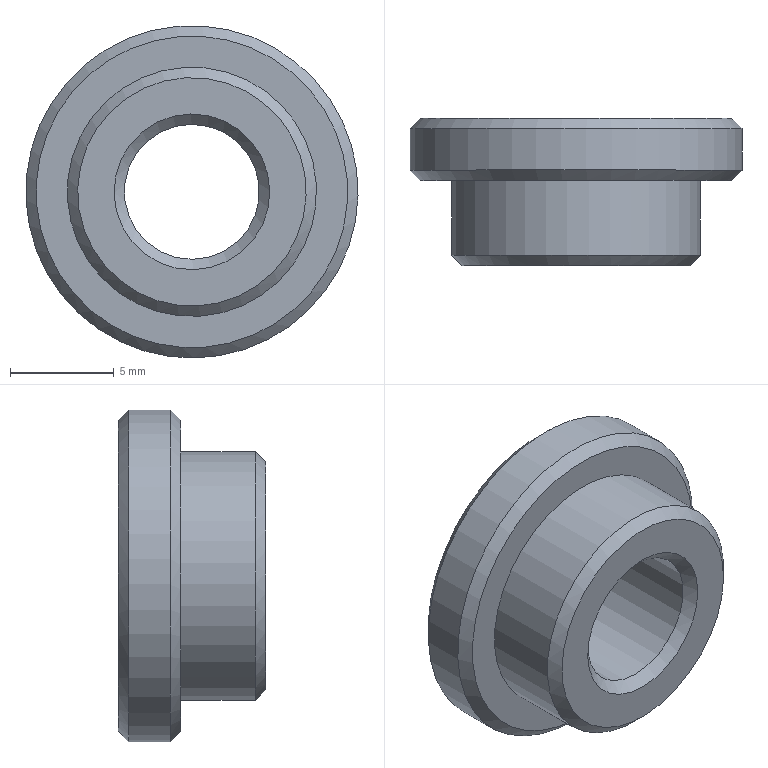Component | NX | BAFFLE | 1 solid | 10 faces | box 16 x 7.1 x 16 mm | volume 812 mm3 | cone 4 | plane 3 | cylinder 3 | commonest cylinder face diameters 16 x1 12 x1 6.5 x1
STEP:
#1=CARTESIAN_POINT('',(0.,0.,0.));
#2=DIRECTION('',(0.,0.,1.));
#3=DIRECTION('',(1.,0.,0.));
#4=AXIS2_PLACEMENT_3D('',#1,#2,#3);
#5=CARTESIAN_POINT('',(68.42,-2.,57.169));
#6=VERTEX_POINT('',#5);
#7=CARTESIAN_POINT('',(70.228,-2.,49.89));
#8=DIRECTION('',(0.,-1.,0.));
#9=DIRECTION('',(-0.2411,0.,0.9705));
#10=AXIS2_PLACEMENT_3D('',#7,#8,#9);
#11=CIRCLE('',#10,7.5);
#12=CARTESIAN_POINT('',(70.228,-2.,49.89));
#13=DIRECTION('',(0.,1.,0.));
#14=DIRECTION('',(-0.2411,0.,0.9705));
#15=AXIS2_PLACEMENT_3D('',#12,#13,#14);
#16=PLANE('',#15);
#17=CARTESIAN_POINT('',(7.5,0.));
#18=CARTESIAN_POINT('',(7.5,-12.99));
#19=CARTESIAN_POINT('',(-3.75,-6.495));
#20=CARTESIAN_POINT('',(-15.,-0.));
#21=CARTESIAN_POINT('',(-3.75,6.495));
#22=CARTESIAN_POINT('',(7.5,12.99));
#23=CARTESIAN_POINT('',(7.5,0.));
#24=(BOUNDED_CURVE()B_SPLINE_CURVE(2,(#17,#18,#19,#20,#21,#22,#23),.UNSPECIFIED.,.T.,.F.)B_SPLINE_CURVE_WITH_KNOTS((1,2,2,2,2,1),(-2.094,0.,2.094,4.189,6.283,8.378),.UNSPECIFIED.)CURVE()GEOMETRIC_REPRESENTATION_ITEM()RATIONAL_B_SPLINE_CURVE((1.,0.5,1.,0.5,1.,0.5,1.))REPRESENTATION_ITEM(''));
#25=(GEOMETRIC_REPRESENTATION_CONTEXT(2)PARAMETRIC_REPRESENTATION_CONTEXT()REPRESENTATION_CONTEXT('',''));
#26=DEFINITIONAL_REPRESENTATION('',(#24),#25);
#27=PCURVE('',#16,#26);
#28=CARTESIAN_POINT('',(70.228,-1.5,49.89));
#29=DIRECTION('',(0.,1.,0.));
#30=DIRECTION('',(-0.2411,0.,0.9705));
#31=AXIS2_PLACEMENT_3D('',#28,#29,#30);
#32=CONICAL_SURFACE('',#31,8.,0.7854);
#33=CARTESIAN_POINT('',(6.283,-0.5));
#34=DIRECTION('',(-1.,0.));
#35=VECTOR('',#34,1.);
#36=LINE('',#33,#35);
#37=(GEOMETRIC_REPRESENTATION_CONTEXT(2)PARAMETRIC_REPRESENTATION_CONTEXT()REPRESENTATION_CONTEXT('',''));
#38=DEFINITIONAL_REPRESENTATION('',(#36),#37);
#39=PCURVE('',#32,#38);
#40=SURFACE_CURVE('',#11,(#27,#39),.PCURVE_S1.);
#41=EDGE_CURVE('',#6,#6,#40,.T.);
#42=ORIENTED_EDGE('',*,*,#41,.T.);
#43=EDGE_LOOP('',(#42));
#44=FACE_BOUND('',#43,.T.);
#45=CARTESIAN_POINT('',(68.781,-2.,55.713));
#46=VERTEX_POINT('',#45);
#47=CARTESIAN_POINT('',(70.228,-2.,49.89));
#48=DIRECTION('',(0.,-1.,0.));
#49=DIRECTION('',(-0.2411,0.,0.9705));
#50=AXIS2_PLACEMENT_3D('',#47,#48,#49);
#51=CIRCLE('',#50,6.);
#52=CARTESIAN_POINT('',(6.,0.));
#53=CARTESIAN_POINT('',(6.,-10.392));
#54=CARTESIAN_POINT('',(-3.,-5.196));
#55=CARTESIAN_POINT('',(-12.,-0.));
#56=CARTESIAN_POINT('',(-3.,5.196));
#57=CARTESIAN_POINT('',(6.,10.392));
#58=CARTESIAN_POINT('',(6.,0.));
#59=(BOUNDED_CURVE()B_SPLINE_CURVE(2,(#52,#53,#54,#55,#56,#57,#58),.UNSPECIFIED.,.T.,.F.)B_SPLINE_CURVE_WITH_KNOTS((1,2,2,2,2,1),(-2.094,0.,2.094,4.189,6.283,8.378),.UNSPECIFIED.)CURVE()GEOMETRIC_REPRESENTATION_ITEM()RATIONAL_B_SPLINE_CURVE((1.,0.5,1.,0.5,1.,0.5,1.))REPRESENTATION_ITEM(''));
#60=(GEOMETRIC_REPRESENTATION_CONTEXT(2)PARAMETRIC_REPRESENTATION_CONTEXT()REPRESENTATION_CONTEXT('',''));
#61=DEFINITIONAL_REPRESENTATION('',(#59),#60);
#62=PCURVE('',#16,#61);
#63=CARTESIAN_POINT('',(70.228,-6.1,49.89));
#64=DIRECTION('',(0.,1.,0.));
#65=DIRECTION('',(-0.2411,0.,0.9705));
#66=AXIS2_PLACEMENT_3D('',#63,#64,#65);
#67=CYLINDRICAL_SURFACE('',#66,6.);
#68=CARTESIAN_POINT('',(6.283,4.1));
#69=DIRECTION('',(-1.,0.));
#70=VECTOR('',#69,1.);
#71=LINE('',#68,#70);
#72=(GEOMETRIC_REPRESENTATION_CONTEXT(2)PARAMETRIC_REPRESENTATION_CONTEXT()REPRESENTATION_CONTEXT('',''));
#73=DEFINITIONAL_REPRESENTATION('',(#71),#72);
#74=PCURVE('',#67,#73);
#75=SURFACE_CURVE('',#51,(#62,#74),.PCURVE_S1.);
#76=EDGE_CURVE('',#46,#46,#75,.T.);
#77=ORIENTED_EDGE('',*,*,#76,.F.);
#78=EDGE_LOOP('',(#77));
#79=FACE_BOUND('',#78,.T.);
#80=ADVANCED_FACE('',(#44,#79),#16,.F.);
#81=CARTESIAN_POINT('',(68.299,0.5,57.654));
#82=VERTEX_POINT('',#81);
#83=CARTESIAN_POINT('',(70.228,0.5,49.89));
#84=DIRECTION('',(0.,-1.,0.));
#85=DIRECTION('',(-0.2411,0.,0.9705));
#86=AXIS2_PLACEMENT_3D('',#83,#84,#85);
#87=CIRCLE('',#86,8.);
#88=CARTESIAN_POINT('',(70.228,1.,49.89));
#89=DIRECTION('',(0.,-1.,0.));
#90=DIRECTION('',(0.2411,0.,-0.9705));
#91=AXIS2_PLACEMENT_3D('',#88,#89,#90);
#92=CYLINDRICAL_SURFACE('',#91,8.);
#93=CARTESIAN_POINT('',(3.142,0.5));
#94=DIRECTION('',(1.,0.));
#95=VECTOR('',#94,1.);
#96=LINE('',#93,#95);
#97=(GEOMETRIC_REPRESENTATION_CONTEXT(2)PARAMETRIC_REPRESENTATION_CONTEXT()REPRESENTATION_CONTEXT('',''));
#98=DEFINITIONAL_REPRESENTATION('',(#96),#97);
#99=PCURVE('',#92,#98);
#100=CARTESIAN_POINT('',(70.228,1.,49.89));
#101=DIRECTION('',(0.,-1.,0.));
#102=DIRECTION('',(0.2411,0.,-0.9705));
#103=AXIS2_PLACEMENT_3D('',#100,#101,#102);
#104=CONICAL_SURFACE('',#103,7.5,0.7854);
#105=CARTESIAN_POINT('',(3.142,0.5));
#106=DIRECTION('',(1.,0.));
#107=VECTOR('',#106,1.);
#108=LINE('',#105,#107);
#109=(GEOMETRIC_REPRESENTATION_CONTEXT(2)PARAMETRIC_REPRESENTATION_CONTEXT()REPRESENTATION_CONTEXT('',''));
#110=DEFINITIONAL_REPRESENTATION('',(#108),#109);
#111=PCURVE('',#104,#110);
#112=SURFACE_CURVE('',#87,(#99,#111),.PCURVE_S1.);
#113=EDGE_CURVE('',#82,#82,#112,.T.);
#114=ORIENTED_EDGE('',*,*,#113,.T.);
#115=CARTESIAN_POINT('',(68.299,-1.5,57.654));
#116=VERTEX_POINT('',#115);
#117=CARTESIAN_POINT('',(68.299,0.5,57.654));
#118=CARTESIAN_POINT('',(68.299,-1.5,57.654));
#119=B_SPLINE_CURVE_WITH_KNOTS('',1,(#117,#118),.UNSPECIFIED.,.F.,.F.,(2,2),(0.5,2.5),.PIECEWISE_BEZIER_KNOTS.);
#120=CARTESIAN_POINT('',(9.425,0.));
#121=DIRECTION('',(0.,1.));
#122=VECTOR('',#121,1.);
#123=LINE('',#120,#122);
#124=(GEOMETRIC_REPRESENTATION_CONTEXT(2)PARAMETRIC_REPRESENTATION_CONTEXT()REPRESENTATION_CONTEXT('',''));
#125=DEFINITIONAL_REPRESENTATION('',(#123),#124);
#126=PCURVE('',#92,#125);
#127=CARTESIAN_POINT('',(3.142,0.));
#128=DIRECTION('',(0.,1.));
#129=VECTOR('',#128,1.);
#130=LINE('',#127,#129);
#131=(GEOMETRIC_REPRESENTATION_CONTEXT(2)PARAMETRIC_REPRESENTATION_CONTEXT()REPRESENTATION_CONTEXT('',''));
#132=DEFINITIONAL_REPRESENTATION('',(#130),#131);
#133=PCURVE('',#92,#132);
#134=SEAM_CURVE('',#119,(#126,#133),.PCURVE_S1.);
#135=EDGE_CURVE('',#82,#116,#134,.T.);
#136=ORIENTED_EDGE('',*,*,#135,.T.);
#137=CARTESIAN_POINT('',(70.228,-1.5,49.89));
#138=DIRECTION('',(0.,1.,0.));
#139=DIRECTION('',(-0.2411,0.,0.9705));
#140=AXIS2_PLACEMENT_3D('',#137,#138,#139);
#141=CIRCLE('',#140,8.);
#142=CARTESIAN_POINT('',(9.425,2.5));
#143=DIRECTION('',(-1.,0.));
#144=VECTOR('',#143,1.);
#145=LINE('',#142,#144);
#146=(GEOMETRIC_REPRESENTATION_CONTEXT(2)PARAMETRIC_REPRESENTATION_CONTEXT()REPRESENTATION_CONTEXT('',''));
#147=DEFINITIONAL_REPRESENTATION('',(#145),#146);
#148=PCURVE('',#92,#147);
#149=CARTESIAN_POINT('',(0.,0.));
#150=DIRECTION('',(1.,0.));
#151=VECTOR('',#150,1.);
#152=LINE('',#149,#151);
#153=(GEOMETRIC_REPRESENTATION_CONTEXT(2)PARAMETRIC_REPRESENTATION_CONTEXT()REPRESENTATION_CONTEXT('',''));
#154=DEFINITIONAL_REPRESENTATION('',(#152),#153);
#155=PCURVE('',#32,#154);
#156=SURFACE_CURVE('',#141,(#148,#155),.PCURVE_S1.);
#157=EDGE_CURVE('',#116,#116,#156,.T.);
#158=ORIENTED_EDGE('',*,*,#157,.T.);
#159=ORIENTED_EDGE('',*,*,#135,.F.);
#160=EDGE_LOOP('',(#114,#136,#158,#159));
#161=FACE_BOUND('',#160,.T.);
#162=ADVANCED_FACE('',(#161),#92,.T.);
#163=CARTESIAN_POINT('',(68.42,1.,57.169));
#164=VERTEX_POINT('',#163);
#165=CARTESIAN_POINT('',(70.228,1.,49.89));
#166=DIRECTION('',(0.,1.,0.));
#167=DIRECTION('',(-0.2411,0.,0.9705));
#168=AXIS2_PLACEMENT_3D('',#165,#166,#167);
#169=CIRCLE('',#168,7.5);
#170=CARTESIAN_POINT('',(70.228,1.,49.89));
#171=DIRECTION('',(0.,1.,0.));
#172=DIRECTION('',(-0.2411,0.,0.9705));
#173=AXIS2_PLACEMENT_3D('',#170,#171,#172);
#174=PLANE('',#173);
#175=CARTESIAN_POINT('',(0.,0.));
#176=DIRECTION('',(1.,0.));
#177=AXIS2_PLACEMENT_2D('',#175,#176);
#178=CIRCLE('',#177,7.5);
#179=(GEOMETRIC_REPRESENTATION_CONTEXT(2)PARAMETRIC_REPRESENTATION_CONTEXT()REPRESENTATION_CONTEXT('',''));
#180=DEFINITIONAL_REPRESENTATION('',(#178),#179);
#181=PCURVE('',#174,#180);
#182=CARTESIAN_POINT('',(9.425,0.));
#183=DIRECTION('',(-1.,0.));
#184=VECTOR('',#183,1.);
#185=LINE('',#182,#184);
#186=(GEOMETRIC_REPRESENTATION_CONTEXT(2)PARAMETRIC_REPRESENTATION_CONTEXT()REPRESENTATION_CONTEXT('',''));
#187=DEFINITIONAL_REPRESENTATION('',(#185),#186);
#188=PCURVE('',#104,#187);
#189=SURFACE_CURVE('',#169,(#181,#188),.PCURVE_S1.);
#190=EDGE_CURVE('',#164,#164,#189,.T.);
#191=ORIENTED_EDGE('',*,*,#190,.T.);
#192=EDGE_LOOP('',(#191));
#193=FACE_BOUND('',#192,.T.);
#194=CARTESIAN_POINT('',(69.444,1.,53.044));
#195=VERTEX_POINT('',#194);
#196=CARTESIAN_POINT('',(70.228,1.,49.89));
#197=DIRECTION('',(0.,1.,0.));
#198=DIRECTION('',(-0.2411,0.,0.9705));
#199=AXIS2_PLACEMENT_3D('',#196,#197,#198);
#200=CIRCLE('',#199,3.25);
#201=CARTESIAN_POINT('',(0.,0.));
#202=DIRECTION('',(1.,-0.));
#203=AXIS2_PLACEMENT_2D('',#201,#202);
#204=CIRCLE('',#203,3.25);
#205=(GEOMETRIC_REPRESENTATION_CONTEXT(2)PARAMETRIC_REPRESENTATION_CONTEXT()REPRESENTATION_CONTEXT('',''));
#206=DEFINITIONAL_REPRESENTATION('',(#204),#205);
#207=PCURVE('',#174,#206);
#208=CARTESIAN_POINT('',(70.228,-6.1,49.89));
#209=DIRECTION('',(0.,1.,0.));
#210=DIRECTION('',(-0.2411,0.,0.9705));
#211=AXIS2_PLACEMENT_3D('',#208,#209,#210);
#212=CYLINDRICAL_SURFACE('',#211,3.25);
#213=CARTESIAN_POINT('',(0.,7.1));
#214=DIRECTION('',(1.,0.));
#215=VECTOR('',#214,1.);
#216=LINE('',#213,#215);
#217=(GEOMETRIC_REPRESENTATION_CONTEXT(2)PARAMETRIC_REPRESENTATION_CONTEXT()REPRESENTATION_CONTEXT('',''));
#218=DEFINITIONAL_REPRESENTATION('',(#216),#217);
#219=PCURVE('',#212,#218);
#220=SURFACE_CURVE('',#200,(#207,#219),.PCURVE_S1.);
#221=EDGE_CURVE('',#195,#195,#220,.T.);
#222=ORIENTED_EDGE('',*,*,#221,.F.);
#223=EDGE_LOOP('',(#222));
#224=FACE_BOUND('',#223,.T.);
#225=ADVANCED_FACE('',(#193,#224),#174,.T.);
#226=CARTESIAN_POINT('',(71.674,-5.6,44.067));
#227=VERTEX_POINT('',#226);
#228=CARTESIAN_POINT('',(68.781,-5.6,55.713));
#229=VERTEX_POINT('',#228);
#230=CARTESIAN_POINT('',(70.228,-5.6,49.89));
#231=DIRECTION('',(0.,1.,0.));
#232=DIRECTION('',(0.2411,0.,-0.9705));
#233=AXIS2_PLACEMENT_3D('',#230,#231,#232);
#234=CIRCLE('',#233,6.);
#235=CARTESIAN_POINT('',(3.142,0.5));
#236=DIRECTION('',(1.,0.));
#237=VECTOR('',#236,1.);
#238=LINE('',#235,#237);
#239=(GEOMETRIC_REPRESENTATION_CONTEXT(2)PARAMETRIC_REPRESENTATION_CONTEXT()REPRESENTATION_CONTEXT('',''));
#240=DEFINITIONAL_REPRESENTATION('',(#238),#239);
#241=PCURVE('',#67,#240);
#242=CARTESIAN_POINT('',(70.228,-6.1,49.89));
#243=DIRECTION('',(0.,1.,0.));
#244=DIRECTION('',(-0.2411,0.,0.9705));
#245=AXIS2_PLACEMENT_3D('',#242,#243,#244);
#246=CONICAL_SURFACE('',#245,5.5,0.7854);
#247=CARTESIAN_POINT('',(3.142,0.5));
#248=DIRECTION('',(1.,-0.));
#249=VECTOR('',#248,1.);
#250=LINE('',#247,#249);
#251=(GEOMETRIC_REPRESENTATION_CONTEXT(2)PARAMETRIC_REPRESENTATION_CONTEXT()REPRESENTATION_CONTEXT('',''));
#252=DEFINITIONAL_REPRESENTATION('',(#250),#251);
#253=PCURVE('',#246,#252);
#254=SURFACE_CURVE('',#234,(#241,#253),.PCURVE_S1.);
#255=EDGE_CURVE('',#227,#229,#254,.T.);
#256=ORIENTED_EDGE('',*,*,#255,.T.);
#257=CARTESIAN_POINT('',(68.781,-5.6,55.713));
#258=CARTESIAN_POINT('',(68.781,-2.,55.713));
#259=B_SPLINE_CURVE_WITH_KNOTS('',1,(#257,#258),.UNSPECIFIED.,.F.,.F.,(2,2),(0.5,4.1),.PIECEWISE_BEZIER_KNOTS.);
#260=CARTESIAN_POINT('',(6.283,0.));
#261=DIRECTION('',(0.,1.));
#262=VECTOR('',#261,1.);
#263=LINE('',#260,#262);
#264=(GEOMETRIC_REPRESENTATION_CONTEXT(2)PARAMETRIC_REPRESENTATION_CONTEXT()REPRESENTATION_CONTEXT('',''));
#265=DEFINITIONAL_REPRESENTATION('',(#263),#264);
#266=PCURVE('',#67,#265);
#267=CARTESIAN_POINT('',(0.,0.));
#268=DIRECTION('',(0.,1.));
#269=VECTOR('',#268,1.);
#270=LINE('',#267,#269);
#271=(GEOMETRIC_REPRESENTATION_CONTEXT(2)PARAMETRIC_REPRESENTATION_CONTEXT()REPRESENTATION_CONTEXT('',''));
#272=DEFINITIONAL_REPRESENTATION('',(#270),#271);
#273=PCURVE('',#67,#272);
#274=SEAM_CURVE('',#259,(#266,#273),.PCURVE_S1.);
#275=EDGE_CURVE('',#229,#46,#274,.T.);
#276=ORIENTED_EDGE('',*,*,#275,.T.);
#277=ORIENTED_EDGE('',*,*,#76,.T.);
#278=ORIENTED_EDGE('',*,*,#275,.F.);
#279=CARTESIAN_POINT('',(70.228,-5.6,49.89));
#280=DIRECTION('',(0.,1.,0.));
#281=DIRECTION('',(0.2411,0.,-0.9705));
#282=AXIS2_PLACEMENT_3D('',#279,#280,#281);
#283=CIRCLE('',#282,6.);
#284=CARTESIAN_POINT('',(-3.142,0.5));
#285=DIRECTION('',(1.,0.));
#286=VECTOR('',#285,1.);
#287=LINE('',#284,#286);
#288=(GEOMETRIC_REPRESENTATION_CONTEXT(2)PARAMETRIC_REPRESENTATION_CONTEXT()REPRESENTATION_CONTEXT('',''));
#289=DEFINITIONAL_REPRESENTATION('',(#287),#288);
#290=PCURVE('',#67,#289);
#291=CARTESIAN_POINT('',(3.142,0.5));
#292=DIRECTION('',(1.,0.));
#293=VECTOR('',#292,1.);
#294=LINE('',#291,#293);
#295=(GEOMETRIC_REPRESENTATION_CONTEXT(2)PARAMETRIC_REPRESENTATION_CONTEXT()REPRESENTATION_CONTEXT('',''));
#296=DEFINITIONAL_REPRESENTATION('',(#294),#295);
#297=PCURVE('',#246,#296);
#298=SURFACE_CURVE('',#283,(#290,#297),.PCURVE_S1.);
#299=EDGE_CURVE('',#229,#227,#298,.T.);
#300=ORIENTED_EDGE('',*,*,#299,.T.);
#301=EDGE_LOOP('',(#256,#276,#277,#278,#300));
#302=FACE_BOUND('',#301,.T.);
#303=ADVANCED_FACE('',(#302),#67,.T.);
#304=CARTESIAN_POINT('',(69.444,-5.6,53.044));
#305=VERTEX_POINT('',#304);
#306=CARTESIAN_POINT('',(71.011,-5.6,46.736));
#307=VERTEX_POINT('',#306);
#308=CARTESIAN_POINT('',(70.228,-5.6,49.89));
#309=DIRECTION('',(0.,-1.,0.));
#310=DIRECTION('',(0.2411,0.,-0.9705));
#311=AXIS2_PLACEMENT_3D('',#308,#309,#310);
#312=CIRCLE('',#311,3.25);
#313=CARTESIAN_POINT('',(9.425,0.5));
#314=DIRECTION('',(-1.,0.));
#315=VECTOR('',#314,1.);
#316=LINE('',#313,#315);
#317=(GEOMETRIC_REPRESENTATION_CONTEXT(2)PARAMETRIC_REPRESENTATION_CONTEXT()REPRESENTATION_CONTEXT('',''));
#318=DEFINITIONAL_REPRESENTATION('',(#316),#317);
#319=PCURVE('',#212,#318);
#320=CARTESIAN_POINT('',(70.228,-6.1,49.89));
#321=DIRECTION('',(0.,-1.,0.));
#322=DIRECTION('',(0.2411,0.,-0.9705));
#323=AXIS2_PLACEMENT_3D('',#320,#321,#322);
#324=CONICAL_SURFACE('',#323,3.75,0.7854);
#325=CARTESIAN_POINT('',(0.,-0.5));
#326=DIRECTION('',(1.,-0.));
#327=VECTOR('',#326,1.);
#328=LINE('',#325,#327);
#329=(GEOMETRIC_REPRESENTATION_CONTEXT(2)PARAMETRIC_REPRESENTATION_CONTEXT()REPRESENTATION_CONTEXT('',''));
#330=DEFINITIONAL_REPRESENTATION('',(#328),#329);
#331=PCURVE('',#324,#330);
#332=SURFACE_CURVE('',#312,(#319,#331),.PCURVE_S1.);
#333=EDGE_CURVE('',#305,#307,#332,.T.);
#334=ORIENTED_EDGE('',*,*,#333,.F.);
#335=CARTESIAN_POINT('',(69.444,-5.6,53.044));
#336=CARTESIAN_POINT('',(69.444,1.,53.044));
#337=B_SPLINE_CURVE_WITH_KNOTS('',1,(#335,#336),.UNSPECIFIED.,.F.,.F.,(2,2),(0.5,7.1),.PIECEWISE_BEZIER_KNOTS.);
#338=CARTESIAN_POINT('',(6.283,0.));
#339=DIRECTION('',(0.,1.));
#340=VECTOR('',#339,1.);
#341=LINE('',#338,#340);
#342=(GEOMETRIC_REPRESENTATION_CONTEXT(2)PARAMETRIC_REPRESENTATION_CONTEXT()REPRESENTATION_CONTEXT('',''));
#343=DEFINITIONAL_REPRESENTATION('',(#341),#342);
#344=PCURVE('',#212,#343);
#345=CARTESIAN_POINT('',(0.,0.));
#346=DIRECTION('',(0.,1.));
#347=VECTOR('',#346,1.);
#348=LINE('',#345,#347);
#349=(GEOMETRIC_REPRESENTATION_CONTEXT(2)PARAMETRIC_REPRESENTATION_CONTEXT()REPRESENTATION_CONTEXT('',''));
#350=DEFINITIONAL_REPRESENTATION('',(#348),#349);
#351=PCURVE('',#212,#350);
#352=SEAM_CURVE('',#337,(#344,#351),.PCURVE_S1.);
#353=EDGE_CURVE('',#305,#195,#352,.T.);
#354=ORIENTED_EDGE('',*,*,#353,.T.);
#355=ORIENTED_EDGE('',*,*,#221,.F.);
#356=ORIENTED_EDGE('',*,*,#353,.F.);
#357=CARTESIAN_POINT('',(70.228,-5.6,49.89));
#358=DIRECTION('',(0.,-1.,0.));
#359=DIRECTION('',(0.2411,0.,-0.9705));
#360=AXIS2_PLACEMENT_3D('',#357,#358,#359);
#361=CIRCLE('',#360,3.25);
#362=CARTESIAN_POINT('',(3.142,0.5));
#363=DIRECTION('',(-1.,0.));
#364=VECTOR('',#363,1.);
#365=LINE('',#362,#364);
#366=(GEOMETRIC_REPRESENTATION_CONTEXT(2)PARAMETRIC_REPRESENTATION_CONTEXT()REPRESENTATION_CONTEXT('',''));
#367=DEFINITIONAL_REPRESENTATION('',(#365),#366);
#368=PCURVE('',#212,#367);
#369=CARTESIAN_POINT('',(0.,-0.5));
#370=DIRECTION('',(1.,0.));
#371=VECTOR('',#370,1.);
#372=LINE('',#369,#371);
#373=(GEOMETRIC_REPRESENTATION_CONTEXT(2)PARAMETRIC_REPRESENTATION_CONTEXT()REPRESENTATION_CONTEXT('',''));
#374=DEFINITIONAL_REPRESENTATION('',(#372),#373);
#375=PCURVE('',#324,#374);
#376=SURFACE_CURVE('',#361,(#368,#375),.PCURVE_S1.);
#377=EDGE_CURVE('',#307,#305,#376,.T.);
#378=ORIENTED_EDGE('',*,*,#377,.F.);
#379=EDGE_LOOP('',(#334,#354,#355,#356,#378));
#380=FACE_BOUND('',#379,.F.);
#381=ADVANCED_FACE('',(#380),#212,.F.);
#382=CARTESIAN_POINT('',(71.132,-6.1,46.251));
#383=VERTEX_POINT('',#382);
#384=CARTESIAN_POINT('',(70.228,-6.1,49.89));
#385=DIRECTION('',(0.,1.,0.));
#386=DIRECTION('',(0.2411,0.,-0.9705));
#387=AXIS2_PLACEMENT_3D('',#384,#385,#386);
#388=CIRCLE('',#387,3.75);
#389=CARTESIAN_POINT('',(70.228,-6.1,49.89));
#390=DIRECTION('',(0.,-1.,0.));
#391=DIRECTION('',(0.2411,0.,-0.9705));
#392=AXIS2_PLACEMENT_3D('',#389,#390,#391);
#393=PLANE('',#392);
#394=CARTESIAN_POINT('',(3.75,0.));
#395=CARTESIAN_POINT('',(3.75,-6.495));
#396=CARTESIAN_POINT('',(-1.875,-3.248));
#397=CARTESIAN_POINT('',(-7.5,-0.));
#398=CARTESIAN_POINT('',(-1.875,3.248));
#399=CARTESIAN_POINT('',(3.75,6.495));
#400=CARTESIAN_POINT('',(3.75,0.));
#401=(BOUNDED_CURVE()B_SPLINE_CURVE(2,(#394,#395,#396,#397,#398,#399,#400),.UNSPECIFIED.,.T.,.F.)B_SPLINE_CURVE_WITH_KNOTS((1,2,2,2,2,1),(-2.094,0.,2.094,4.189,6.283,8.378),.UNSPECIFIED.)CURVE()GEOMETRIC_REPRESENTATION_ITEM()RATIONAL_B_SPLINE_CURVE((1.,0.5,1.,0.5,1.,0.5,1.))REPRESENTATION_ITEM(''));
#402=(GEOMETRIC_REPRESENTATION_CONTEXT(2)PARAMETRIC_REPRESENTATION_CONTEXT()REPRESENTATION_CONTEXT('',''));
#403=DEFINITIONAL_REPRESENTATION('',(#401),#402);
#404=PCURVE('',#393,#403);
#405=CARTESIAN_POINT('',(6.283,0.));
#406=DIRECTION('',(-1.,0.));
#407=VECTOR('',#406,1.);
#408=LINE('',#405,#407);
#409=(GEOMETRIC_REPRESENTATION_CONTEXT(2)PARAMETRIC_REPRESENTATION_CONTEXT()REPRESENTATION_CONTEXT('',''));
#410=DEFINITIONAL_REPRESENTATION('',(#408),#409);
#411=PCURVE('',#324,#410);
#412=SURFACE_CURVE('',#388,(#404,#411),.PCURVE_S1.);
#413=EDGE_CURVE('',#383,#383,#412,.T.);
#414=ORIENTED_EDGE('',*,*,#413,.T.);
#415=EDGE_LOOP('',(#414));
#416=FACE_BOUND('',#415,.T.);
#417=CARTESIAN_POINT('',(71.554,-6.1,44.552));
#418=VERTEX_POINT('',#417);
#419=CARTESIAN_POINT('',(70.228,-6.1,49.89));
#420=DIRECTION('',(0.,-1.,0.));
#421=DIRECTION('',(0.2411,0.,-0.9705));
#422=AXIS2_PLACEMENT_3D('',#419,#420,#421);
#423=CIRCLE('',#422,5.5);
#424=CARTESIAN_POINT('',(0.,0.));
#425=DIRECTION('',(1.,0.));
#426=AXIS2_PLACEMENT_2D('',#424,#425);
#427=CIRCLE('',#426,5.5);
#428=(GEOMETRIC_REPRESENTATION_CONTEXT(2)PARAMETRIC_REPRESENTATION_CONTEXT()REPRESENTATION_CONTEXT('',''));
#429=DEFINITIONAL_REPRESENTATION('',(#427),#428);
#430=PCURVE('',#393,#429);
#431=CARTESIAN_POINT('',(9.425,-0.));
#432=DIRECTION('',(-1.,0.));
#433=VECTOR('',#432,1.);
#434=LINE('',#431,#433);
#435=(GEOMETRIC_REPRESENTATION_CONTEXT(2)PARAMETRIC_REPRESENTATION_CONTEXT()REPRESENTATION_CONTEXT('',''));
#436=DEFINITIONAL_REPRESENTATION('',(#434),#435);
#437=PCURVE('',#246,#436);
#438=SURFACE_CURVE('',#423,(#430,#437),.PCURVE_S1.);
#439=EDGE_CURVE('',#418,#418,#438,.T.);
#440=ORIENTED_EDGE('',*,*,#439,.T.);
#441=EDGE_LOOP('',(#440));
#442=FACE_BOUND('',#441,.T.);
#443=ADVANCED_FACE('',(#416,#442),#393,.T.);
#444=ORIENTED_EDGE('',*,*,#113,.F.);
#445=CARTESIAN_POINT('',(68.42,1.,57.169));
#446=CARTESIAN_POINT('',(68.299,0.5,57.654));
#447=B_SPLINE_CURVE_WITH_KNOTS('',1,(#445,#446),.UNSPECIFIED.,.F.,.F.,(2,2),(0.,0.7071),.PIECEWISE_BEZIER_KNOTS.);
#448=CARTESIAN_POINT('',(3.142,0.));
#449=DIRECTION('',(0.,1.));
#450=VECTOR('',#449,1.);
#451=LINE('',#448,#450);
#452=(GEOMETRIC_REPRESENTATION_CONTEXT(2)PARAMETRIC_REPRESENTATION_CONTEXT()REPRESENTATION_CONTEXT('',''));
#453=DEFINITIONAL_REPRESENTATION('',(#451),#452);
#454=PCURVE('',#104,#453);
#455=CARTESIAN_POINT('',(9.425,0.));
#456=DIRECTION('',(0.,1.));
#457=VECTOR('',#456,1.);
#458=LINE('',#455,#457);
#459=(GEOMETRIC_REPRESENTATION_CONTEXT(2)PARAMETRIC_REPRESENTATION_CONTEXT()REPRESENTATION_CONTEXT('',''));
#460=DEFINITIONAL_REPRESENTATION('',(#458),#459);
#461=PCURVE('',#104,#460);
#462=SEAM_CURVE('',#447,(#454,#461),.PCURVE_S1.);
#463=EDGE_CURVE('',#164,#82,#462,.T.);
#464=ORIENTED_EDGE('',*,*,#463,.F.);
#465=ORIENTED_EDGE('',*,*,#190,.F.);
#466=ORIENTED_EDGE('',*,*,#463,.T.);
#467=EDGE_LOOP('',(#444,#464,#465,#466));
#468=FACE_BOUND('',#467,.T.);
#469=ADVANCED_FACE('',(#468),#104,.T.);
#470=ORIENTED_EDGE('',*,*,#41,.F.);
#471=CARTESIAN_POINT('',(68.42,-2.,57.169));
#472=CARTESIAN_POINT('',(68.299,-1.5,57.654));
#473=B_SPLINE_CURVE_WITH_KNOTS('',1,(#471,#472),.UNSPECIFIED.,.F.,.F.,(2,2),(-0.7071,0.),.PIECEWISE_BEZIER_KNOTS.);
#474=CARTESIAN_POINT('',(6.283,0.));
#475=DIRECTION('',(0.,1.));
#476=VECTOR('',#475,1.);
#477=LINE('',#474,#476);
#478=(GEOMETRIC_REPRESENTATION_CONTEXT(2)PARAMETRIC_REPRESENTATION_CONTEXT()REPRESENTATION_CONTEXT('',''));
#479=DEFINITIONAL_REPRESENTATION('',(#477),#478);
#480=PCURVE('',#32,#479);
#481=CARTESIAN_POINT('',(0.,0.));
#482=DIRECTION('',(0.,1.));
#483=VECTOR('',#482,1.);
#484=LINE('',#481,#483);
#485=(GEOMETRIC_REPRESENTATION_CONTEXT(2)PARAMETRIC_REPRESENTATION_CONTEXT()REPRESENTATION_CONTEXT('',''));
#486=DEFINITIONAL_REPRESENTATION('',(#484),#485);
#487=PCURVE('',#32,#486);
#488=SEAM_CURVE('',#473,(#480,#487),.PCURVE_S1.);
#489=EDGE_CURVE('',#6,#116,#488,.T.);
#490=ORIENTED_EDGE('',*,*,#489,.T.);
#491=ORIENTED_EDGE('',*,*,#157,.F.);
#492=ORIENTED_EDGE('',*,*,#489,.F.);
#493=EDGE_LOOP('',(#470,#490,#491,#492));
#494=FACE_BOUND('',#493,.T.);
#495=ADVANCED_FACE('',(#494),#32,.T.);
#496=ORIENTED_EDGE('',*,*,#255,.F.);
#497=CARTESIAN_POINT('',(71.554,-6.1,44.552));
#498=CARTESIAN_POINT('',(71.674,-5.6,44.067));
#499=B_SPLINE_CURVE_WITH_KNOTS('',1,(#497,#498),.UNSPECIFIED.,.F.,.F.,(2,2),(-0.,0.7071),.PIECEWISE_BEZIER_KNOTS.);
#500=CARTESIAN_POINT('',(3.142,0.));
#501=DIRECTION('',(0.,1.));
#502=VECTOR('',#501,1.);
#503=LINE('',#500,#502);
#504=(GEOMETRIC_REPRESENTATION_CONTEXT(2)PARAMETRIC_REPRESENTATION_CONTEXT()REPRESENTATION_CONTEXT('',''));
#505=DEFINITIONAL_REPRESENTATION('',(#503),#504);
#506=PCURVE('',#246,#505);
#507=CARTESIAN_POINT('',(9.425,0.));
#508=DIRECTION('',(0.,1.));
#509=VECTOR('',#508,1.);
#510=LINE('',#507,#509);
#511=(GEOMETRIC_REPRESENTATION_CONTEXT(2)PARAMETRIC_REPRESENTATION_CONTEXT()REPRESENTATION_CONTEXT('',''));
#512=DEFINITIONAL_REPRESENTATION('',(#510),#511);
#513=PCURVE('',#246,#512);
#514=SEAM_CURVE('',#499,(#506,#513),.PCURVE_S1.);
#515=EDGE_CURVE('',#418,#227,#514,.T.);
#516=ORIENTED_EDGE('',*,*,#515,.F.);
#517=ORIENTED_EDGE('',*,*,#439,.F.);
#518=ORIENTED_EDGE('',*,*,#515,.T.);
#519=ORIENTED_EDGE('',*,*,#299,.F.);
#520=EDGE_LOOP('',(#496,#516,#517,#518,#519));
#521=FACE_BOUND('',#520,.T.);
#522=ADVANCED_FACE('',(#521),#246,.T.);
#523=ORIENTED_EDGE('',*,*,#333,.T.);
#524=CARTESIAN_POINT('',(71.011,-5.6,46.736));
#525=CARTESIAN_POINT('',(71.132,-6.1,46.251));
#526=B_SPLINE_CURVE_WITH_KNOTS('',1,(#524,#525),.UNSPECIFIED.,.F.,.F.,(2,2),(-0.7071,0.),.PIECEWISE_BEZIER_KNOTS.);
#527=CARTESIAN_POINT('',(6.283,0.));
#528=DIRECTION('',(0.,1.));
#529=VECTOR('',#528,1.);
#530=LINE('',#527,#529);
#531=(GEOMETRIC_REPRESENTATION_CONTEXT(2)PARAMETRIC_REPRESENTATION_CONTEXT()REPRESENTATION_CONTEXT('',''));
#532=DEFINITIONAL_REPRESENTATION('',(#530),#531);
#533=PCURVE('',#324,#532);
#534=CARTESIAN_POINT('',(0.,0.));
#535=DIRECTION('',(0.,1.));
#536=VECTOR('',#535,1.);
#537=LINE('',#534,#536);
#538=(GEOMETRIC_REPRESENTATION_CONTEXT(2)PARAMETRIC_REPRESENTATION_CONTEXT()REPRESENTATION_CONTEXT('',''));
#539=DEFINITIONAL_REPRESENTATION('',(#537),#538);
#540=PCURVE('',#324,#539);
#541=SEAM_CURVE('',#526,(#533,#540),.PCURVE_S1.);
#542=EDGE_CURVE('',#307,#383,#541,.T.);
#543=ORIENTED_EDGE('',*,*,#542,.T.);
#544=ORIENTED_EDGE('',*,*,#413,.T.);
#545=ORIENTED_EDGE('',*,*,#542,.F.);
#546=ORIENTED_EDGE('',*,*,#377,.T.);
#547=EDGE_LOOP('',(#523,#543,#544,#545,#546));
#548=FACE_BOUND('',#547,.F.);
#549=ADVANCED_FACE('',(#548),#324,.F.);
#550=CLOSED_SHELL('',(#80,#162,#225,#303,#381,#443,#469,#495,#522,#549));
#551=MANIFOLD_SOLID_BREP('',#550);
#552=(LENGTH_UNIT()NAMED_UNIT(*)SI_UNIT(.MILLI.,.METRE.));
#553=UNCERTAINTY_MEASURE_WITH_UNIT(LENGTH_MEASURE(0.00001),#552,'','');
#554=(NAMED_UNIT(*)PLANE_ANGLE_UNIT()SI_UNIT($,.RADIAN.));
#555=(NAMED_UNIT(*)SI_UNIT($,.STERADIAN.)SOLID_ANGLE_UNIT());
#556=(GEOMETRIC_REPRESENTATION_CONTEXT(3)GLOBAL_UNCERTAINTY_ASSIGNED_CONTEXT((#553))GLOBAL_UNIT_ASSIGNED_CONTEXT((#552,#554,#555))REPRESENTATION_CONTEXT('',''));
#557=ADVANCED_BREP_SHAPE_REPRESENTATION('',(#4,#551),#556);